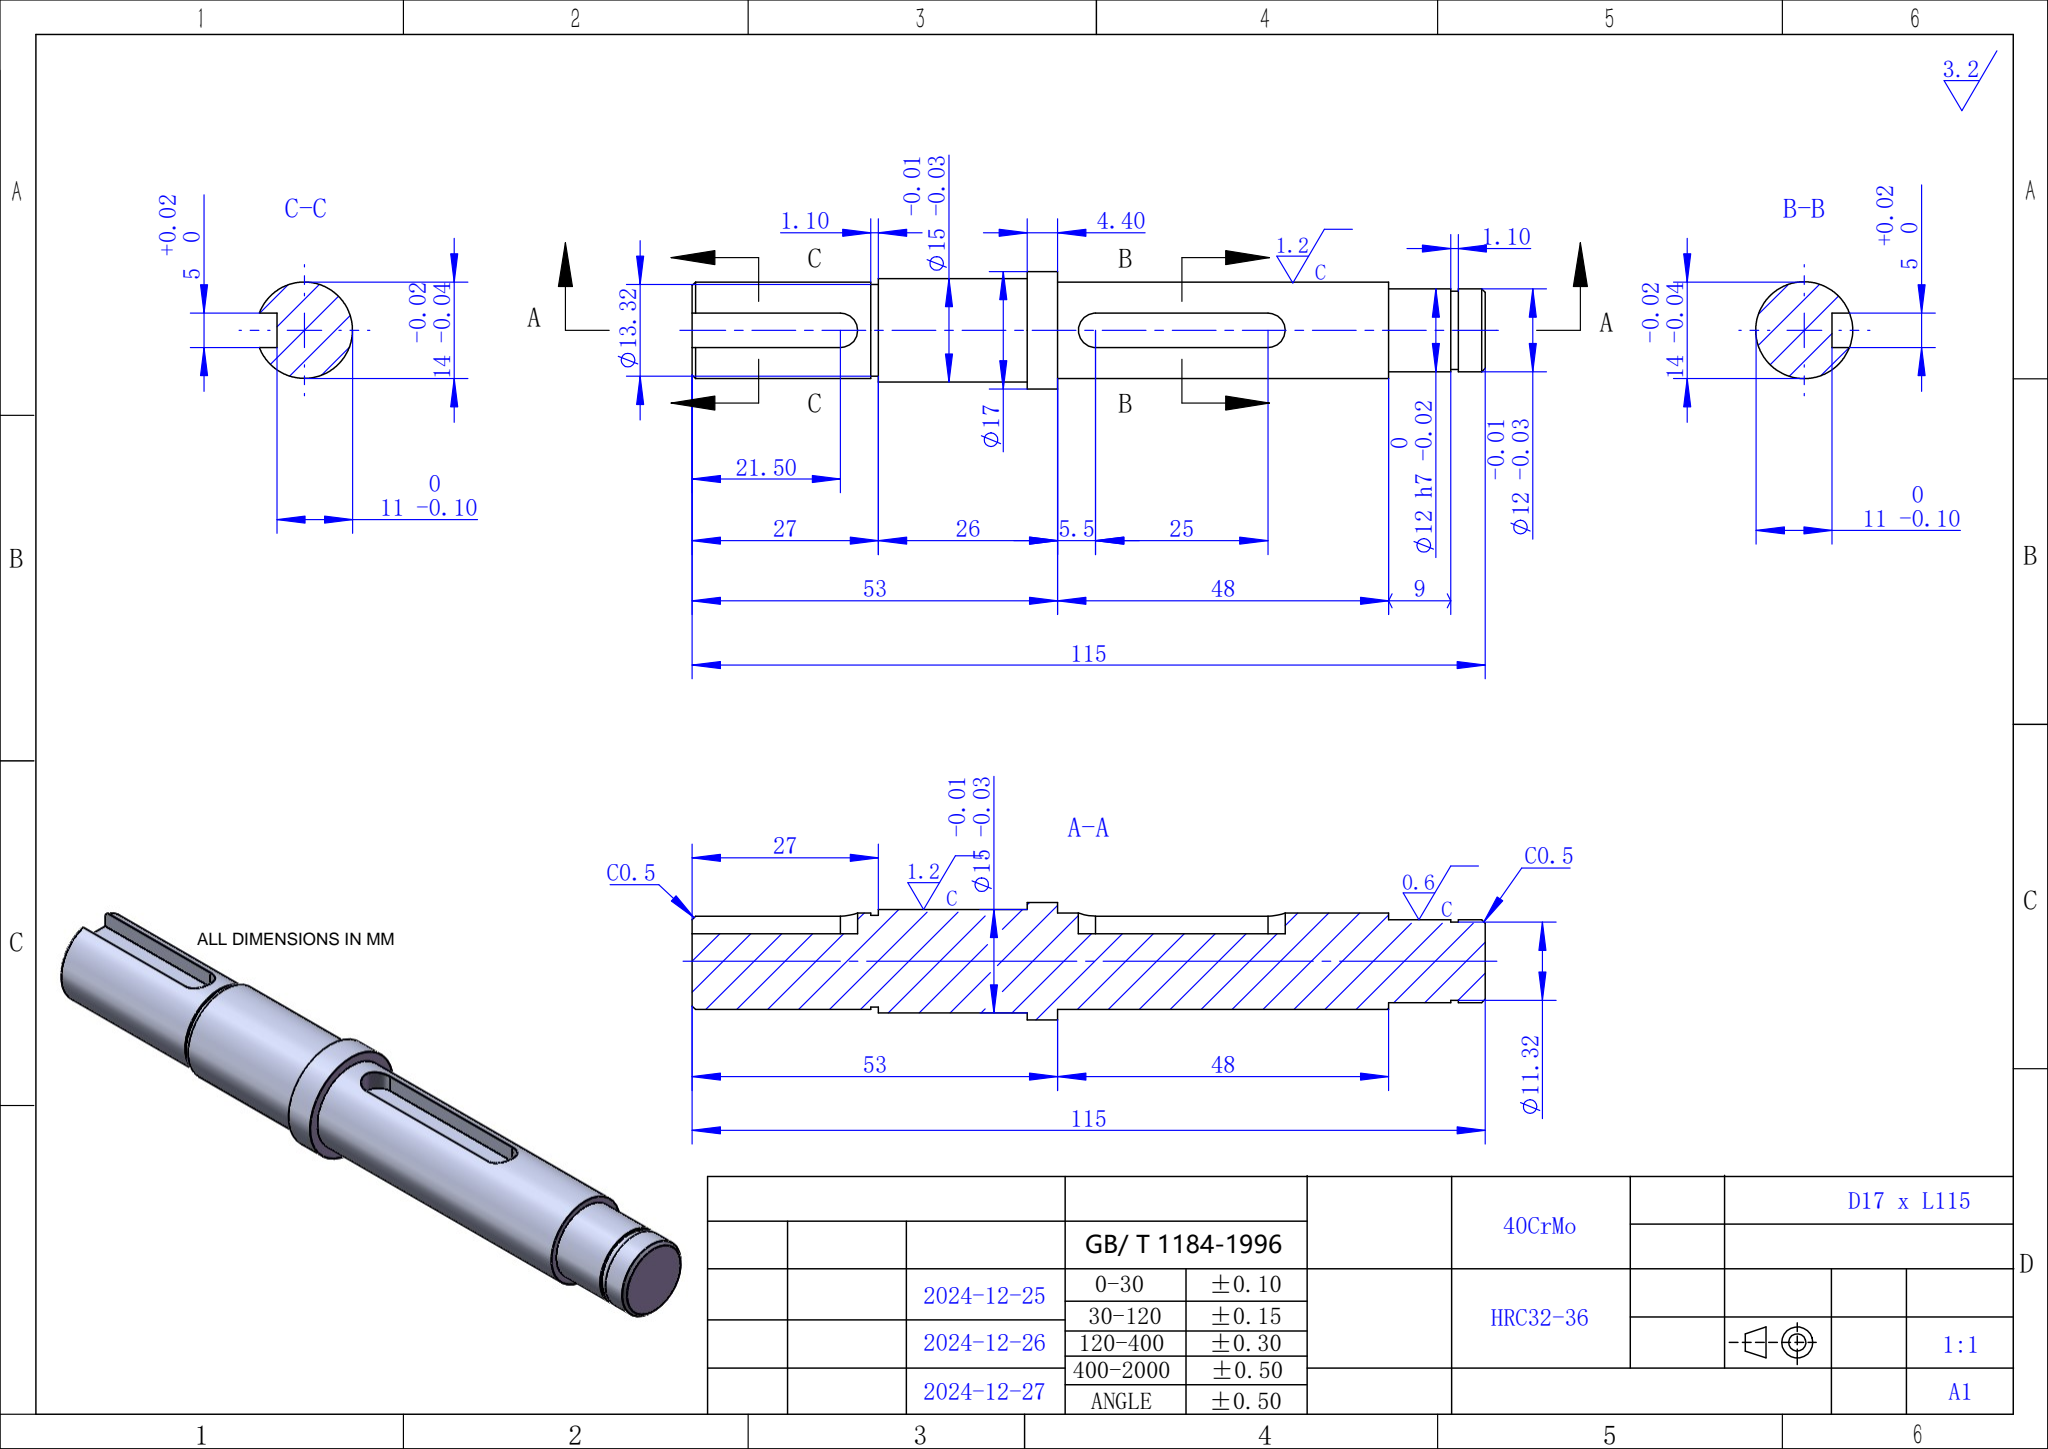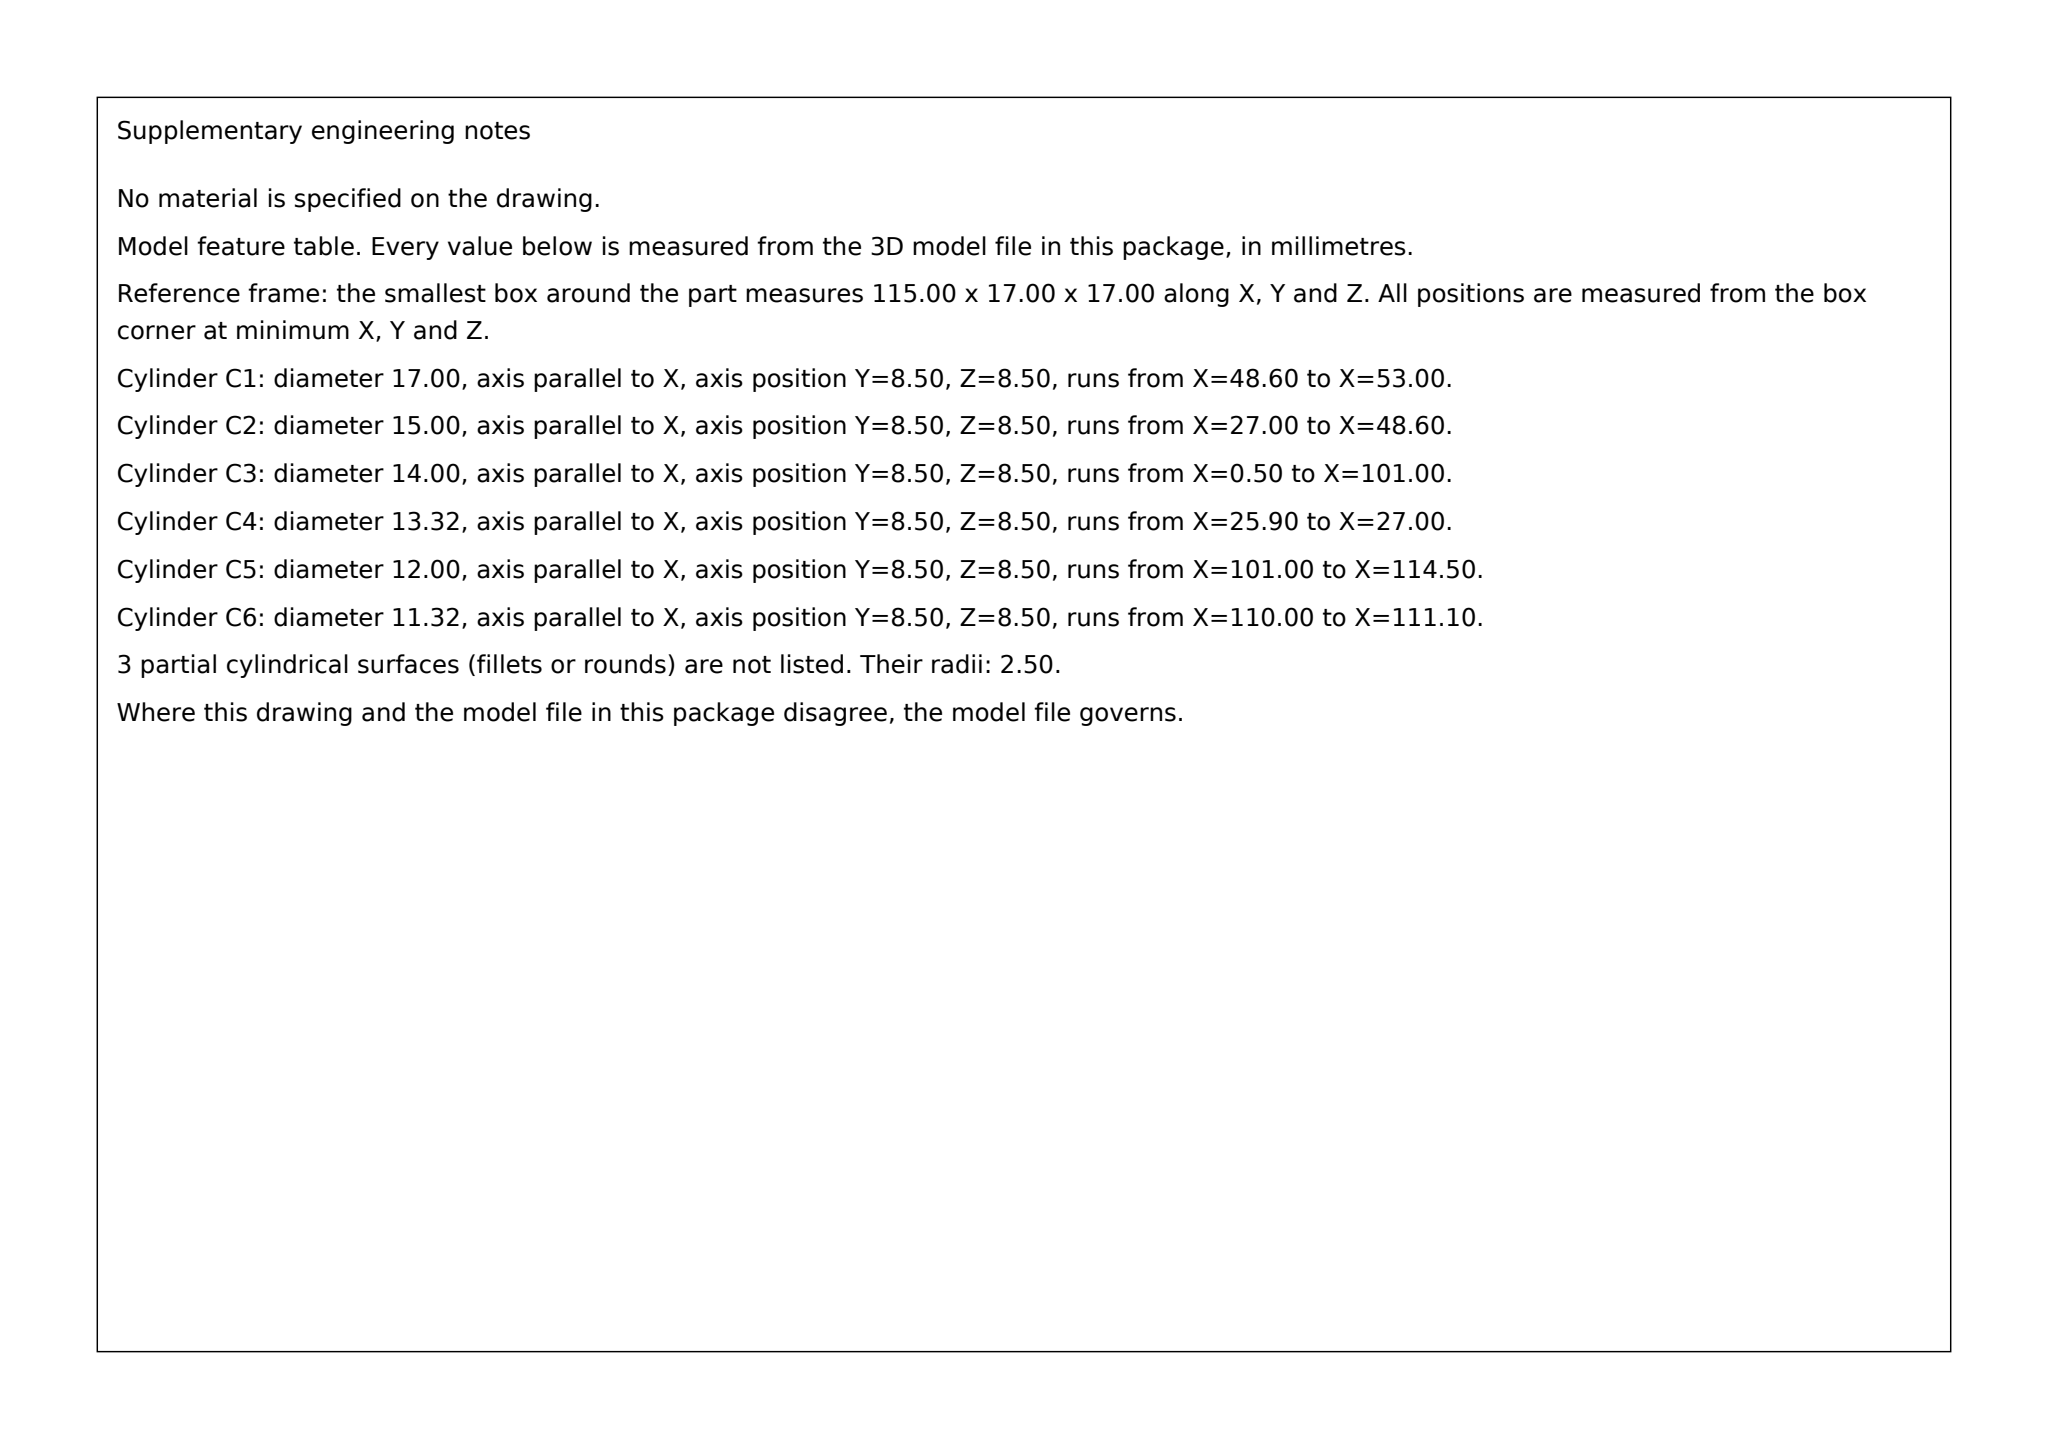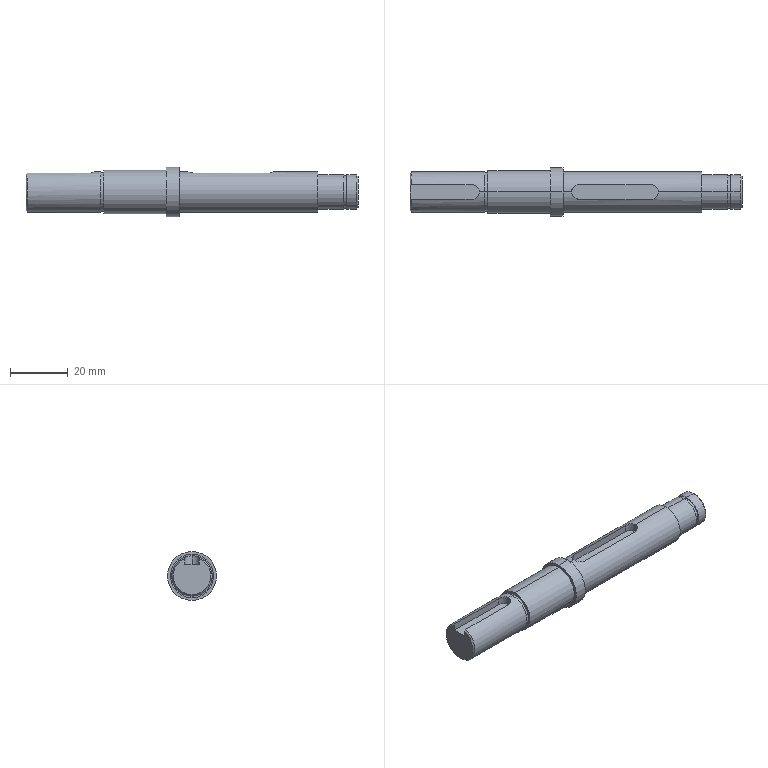Part | SolidWorks | mm | material 40CrMo | 1 solid | 40 faces | box 115 x 17 x 17 mm | volume 17158 mm3 | cylinder 21 | plane 15 | cone 4 | commonest cylinder face diameters 5 x5 12 x4 14 x4 11.32 x2 17 x2 15 x2 13.32 x2
build123d program:
from build123d import *

# Parameters (mm, degrees)
CUT_EXTRUDE1_DEPTH = 3


with BuildPart() as part:
    # Sketch1 → Revolve1 (revolve)
    with BuildSketch(Plane.XY, mode=Mode.PRIVATE) as revolve1_sk:
        Polygon((0, 0), (0, -6.5), (0.5, -7), (25.9, -7), (25.9, -6.66), (27, -6.66), (27, -7.5), (48.6, -7.5), (48.6, -8.5), (53, -8.5), (53, -7), (101, -7), (101, -6), (110, -6), (110, -5.66), (111.1, -5.66), (111.1, -6), (114.5, -6), (115, -5.5), (115, 0), align=None)
    revolve(revolve1_sk.sketch.rotate(Axis((0, 0, 0), (1, 0, 0)), 270), axis=Axis((0, 0, 0), (1, 0, 0)))

    # Sketch3 → Cut-Extrude1 (cut)
    with BuildSketch(Plane.XY.offset(7)):
        with BuildLine():
            Line((0, 2.5), (21.5, 2.5))
            ThreePointArc((21.5, 2.5), (24, 0), (21.5, -2.5))
            Line((21.5, -2.5), (0, -2.5))
            ThreePointArc((0, -2.5), (-2.5, 0), (0, 2.5))
        make_face()
        with BuildLine():
            Line((58.5, 2.5), (83.5, 2.5))
            ThreePointArc((83.5, 2.5), (86, 0), (83.5, -2.5))
            Line((83.5, -2.5), (58.5, -2.5))
            ThreePointArc((58.5, -2.5), (56, 0), (58.5, 2.5))
        make_face()
    extrude(amount=-CUT_EXTRUDE1_DEPTH, mode=Mode.SUBTRACT)


solid = part.part